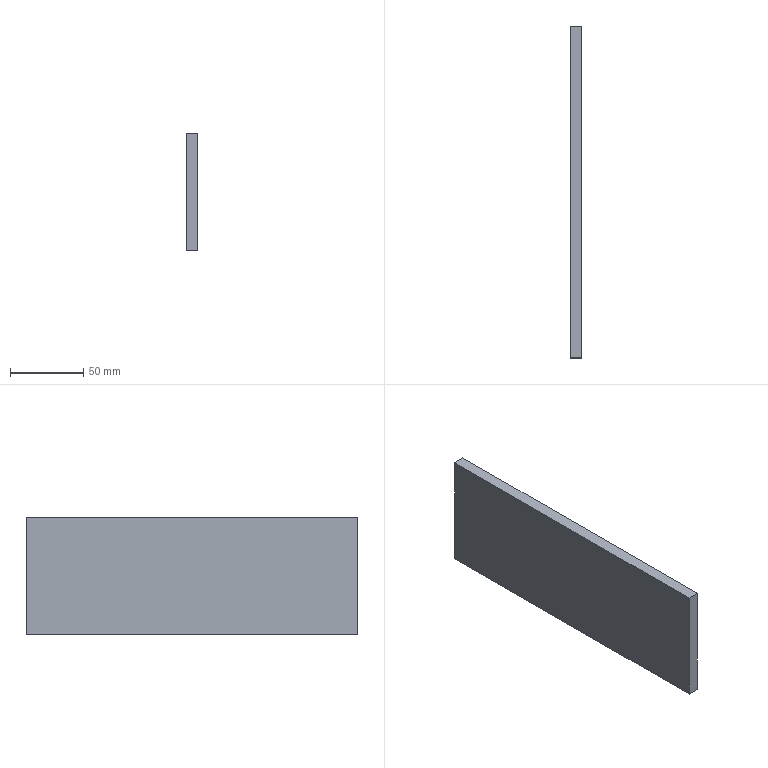Component | SolidWorks | RibPlate1-1 | 1 solid | 6 faces | box 8 x 226 x 80 mm | volume 144640 mm3 | plane 6 | material Plain Carbon Steel
STEP:
#1=CARTESIAN_POINT('',(17.897,53.911,65.555));
#2=VERTEX_POINT('',#1);
#3=CARTESIAN_POINT('',(17.897,53.911,68.704));
#4=VERTEX_POINT('',#3);
#5=CARTESIAN_POINT('',(17.897,53.911,68.704));
#6=DIRECTION('',(0.,-0.,1.));
#7=VECTOR('',#6,39.37);
#8=LINE('',#5,#7);
#9=EDGE_CURVE('',#2,#4,#8,.T.);
#10=ORIENTED_EDGE('',*,*,#9,.F.);
#11=CARTESIAN_POINT('',(17.582,53.911,65.555));
#12=VERTEX_POINT('',#11);
#13=CARTESIAN_POINT('',(17.582,53.911,65.555));
#14=DIRECTION('',(1.,0.,0.));
#15=VECTOR('',#14,39.37);
#16=LINE('',#13,#15);
#17=EDGE_CURVE('',#12,#2,#16,.T.);
#18=ORIENTED_EDGE('',*,*,#17,.F.);
#19=CARTESIAN_POINT('',(17.582,53.911,68.704));
#20=VERTEX_POINT('',#19);
#21=CARTESIAN_POINT('',(17.582,53.911,68.704));
#22=DIRECTION('',(0.,-0.,1.));
#23=VECTOR('',#22,39.37);
#24=LINE('',#21,#23);
#25=EDGE_CURVE('',#12,#20,#24,.T.);
#26=ORIENTED_EDGE('',*,*,#25,.T.);
#27=CARTESIAN_POINT('',(17.582,53.911,68.704));
#28=DIRECTION('',(1.,0.,0.));
#29=VECTOR('',#28,39.37);
#30=LINE('',#27,#29);
#31=EDGE_CURVE('',#20,#4,#30,.T.);
#32=ORIENTED_EDGE('',*,*,#31,.T.);
#33=EDGE_LOOP('',(#10,#18,#26,#32));
#34=FACE_OUTER_BOUND('',#33,.T.);
#35=CARTESIAN_POINT('',(17.582,53.911,68.704));
#36=DIRECTION('',(0.,1.,0.));
#37=DIRECTION('',(-1.,0.,0.));
#38=AXIS2_PLACEMENT_3D('',#35,#36,#37);
#39=PLANE('',#38);
#40=ADVANCED_FACE('',(#34),#39,.T.);
#41=CARTESIAN_POINT('',(17.897,45.014,65.555));
#42=VERTEX_POINT('',#41);
#43=CARTESIAN_POINT('',(17.897,45.014,65.555));
#44=DIRECTION('',(0.,1.,0.));
#45=VECTOR('',#44,39.37);
#46=LINE('',#43,#45);
#47=EDGE_CURVE('',#42,#2,#46,.T.);
#48=ORIENTED_EDGE('',*,*,#47,.F.);
#49=CARTESIAN_POINT('',(17.582,45.014,65.555));
#50=VERTEX_POINT('',#49);
#51=CARTESIAN_POINT('',(17.582,45.014,65.555));
#52=DIRECTION('',(1.,0.,0.));
#53=VECTOR('',#52,39.37);
#54=LINE('',#51,#53);
#55=EDGE_CURVE('',#50,#42,#54,.T.);
#56=ORIENTED_EDGE('',*,*,#55,.F.);
#57=CARTESIAN_POINT('',(17.582,45.014,65.555));
#58=DIRECTION('',(0.,1.,0.));
#59=VECTOR('',#58,39.37);
#60=LINE('',#57,#59);
#61=EDGE_CURVE('',#50,#12,#60,.T.);
#62=ORIENTED_EDGE('',*,*,#61,.T.);
#63=ORIENTED_EDGE('',*,*,#17,.T.);
#64=EDGE_LOOP('',(#48,#56,#62,#63));
#65=FACE_OUTER_BOUND('',#64,.T.);
#66=CARTESIAN_POINT('',(17.582,45.014,65.555));
#67=DIRECTION('',(0.,0.,-1.));
#68=DIRECTION('',(0.,1.,0.));
#69=AXIS2_PLACEMENT_3D('',#66,#67,#68);
#70=PLANE('',#69);
#71=ADVANCED_FACE('',(#65),#70,.T.);
#72=CARTESIAN_POINT('',(17.897,45.014,68.704));
#73=VERTEX_POINT('',#72);
#74=CARTESIAN_POINT('',(17.897,45.014,68.704));
#75=DIRECTION('',(0.,0.,-1.));
#76=VECTOR('',#75,39.37);
#77=LINE('',#74,#76);
#78=EDGE_CURVE('',#73,#42,#77,.T.);
#79=ORIENTED_EDGE('',*,*,#78,.F.);
#80=CARTESIAN_POINT('',(17.582,45.014,68.704));
#81=VERTEX_POINT('',#80);
#82=CARTESIAN_POINT('',(17.582,45.014,68.704));
#83=DIRECTION('',(1.,0.,0.));
#84=VECTOR('',#83,39.37);
#85=LINE('',#82,#84);
#86=EDGE_CURVE('',#81,#73,#85,.T.);
#87=ORIENTED_EDGE('',*,*,#86,.F.);
#88=CARTESIAN_POINT('',(17.582,45.014,68.704));
#89=DIRECTION('',(0.,0.,-1.));
#90=VECTOR('',#89,39.37);
#91=LINE('',#88,#90);
#92=EDGE_CURVE('',#81,#50,#91,.T.);
#93=ORIENTED_EDGE('',*,*,#92,.T.);
#94=ORIENTED_EDGE('',*,*,#55,.T.);
#95=EDGE_LOOP('',(#79,#87,#93,#94));
#96=FACE_OUTER_BOUND('',#95,.T.);
#97=CARTESIAN_POINT('',(17.582,45.014,68.704));
#98=DIRECTION('',(0.,-1.,-0.));
#99=DIRECTION('',(0.,0.,-1.));
#100=AXIS2_PLACEMENT_3D('',#97,#98,#99);
#101=PLANE('',#100);
#102=ADVANCED_FACE('',(#96),#101,.T.);
#103=CARTESIAN_POINT('',(17.897,45.014,68.704));
#104=DIRECTION('',(0.,-1.,-0.));
#105=VECTOR('',#104,39.37);
#106=LINE('',#103,#105);
#107=EDGE_CURVE('',#4,#73,#106,.T.);
#108=ORIENTED_EDGE('',*,*,#107,.F.);
#109=ORIENTED_EDGE('',*,*,#31,.F.);
#110=CARTESIAN_POINT('',(17.582,45.014,68.704));
#111=DIRECTION('',(0.,-1.,-0.));
#112=VECTOR('',#111,39.37);
#113=LINE('',#110,#112);
#114=EDGE_CURVE('',#20,#81,#113,.T.);
#115=ORIENTED_EDGE('',*,*,#114,.T.);
#116=ORIENTED_EDGE('',*,*,#86,.T.);
#117=EDGE_LOOP('',(#108,#109,#115,#116));
#118=FACE_OUTER_BOUND('',#117,.T.);
#119=CARTESIAN_POINT('',(17.582,45.014,68.704));
#120=DIRECTION('',(0.,-0.,1.));
#121=DIRECTION('',(0.,-1.,-0.));
#122=AXIS2_PLACEMENT_3D('',#119,#120,#121);
#123=PLANE('',#122);
#124=ADVANCED_FACE('',(#118),#123,.T.);
#125=ORIENTED_EDGE('',*,*,#25,.F.);
#126=ORIENTED_EDGE('',*,*,#61,.F.);
#127=ORIENTED_EDGE('',*,*,#92,.F.);
#128=ORIENTED_EDGE('',*,*,#114,.F.);
#129=EDGE_LOOP('',(#125,#126,#127,#128));
#130=FACE_OUTER_BOUND('',#129,.T.);
#131=CARTESIAN_POINT('',(17.582,49.134,62.367));
#132=DIRECTION('',(1.,0.,0.));
#133=DIRECTION('',(0.,1.,0.));
#134=AXIS2_PLACEMENT_3D('',#131,#132,#133);
#135=PLANE('',#134);
#136=ADVANCED_FACE('',(#130),#135,.F.);
#137=ORIENTED_EDGE('',*,*,#9,.T.);
#138=ORIENTED_EDGE('',*,*,#107,.T.);
#139=ORIENTED_EDGE('',*,*,#78,.T.);
#140=ORIENTED_EDGE('',*,*,#47,.T.);
#141=EDGE_LOOP('',(#137,#138,#139,#140));
#142=FACE_OUTER_BOUND('',#141,.T.);
#143=CARTESIAN_POINT('',(17.897,49.134,62.367));
#144=DIRECTION('',(1.,0.,0.));
#145=DIRECTION('',(0.,1.,0.));
#146=AXIS2_PLACEMENT_3D('',#143,#144,#145);
#147=PLANE('',#146);
#148=ADVANCED_FACE('',(#142),#147,.T.);
#149=CLOSED_SHELL('',(#40,#71,#102,#124,#136,#148));
#150=MANIFOLD_SOLID_BREP('',#149);
#151=CARTESIAN_POINT('',(0.,0.,0.));
#152=DIRECTION('',(0.,0.,1.));
#153=DIRECTION('',(1.,0.,0.));
#154=AXIS2_PLACEMENT_3D('',#151,#152,#153);
#155=(LENGTH_UNIT()NAMED_UNIT(*)SI_UNIT($,.METRE.));
#156=LENGTH_MEASURE_WITH_UNIT(LENGTH_MEASURE(0.0254),#155);
#157=DIMENSIONAL_EXPONENTS(1.,0.,0.,0.,0.,0.,0.);
#158=(CONVERSION_BASED_UNIT('',#156)LENGTH_UNIT()NAMED_UNIT(#157));
#159=UNCERTAINTY_MEASURE_WITH_UNIT(LENGTH_MEASURE(0.00001),#158,'','');
#160=(NAMED_UNIT(*)PLANE_ANGLE_UNIT()SI_UNIT($,.RADIAN.));
#161=(NAMED_UNIT(*)SI_UNIT($,.STERADIAN.)SOLID_ANGLE_UNIT());
#162=(GEOMETRIC_REPRESENTATION_CONTEXT(3)GLOBAL_UNCERTAINTY_ASSIGNED_CONTEXT((#159))GLOBAL_UNIT_ASSIGNED_CONTEXT((#158,#160,#161))REPRESENTATION_CONTEXT('',''));
#163=ADVANCED_BREP_SHAPE_REPRESENTATION('',(#150,#154),#162);
#164=COLOUR_RGB('',0.7922,0.8196,0.9333);
#165=FILL_AREA_STYLE_COLOUR('',#164);
#166=FILL_AREA_STYLE('',(#165));
#167=SURFACE_STYLE_FILL_AREA(#166);
#168=SURFACE_SIDE_STYLE('',(#167));
#169=SURFACE_STYLE_USAGE(.BOTH.,#168);
#170=PRESENTATION_STYLE_ASSIGNMENT((#169));
#171=STYLED_ITEM('',(#170),#150);
#172=(LENGTH_UNIT()NAMED_UNIT(*)SI_UNIT($,.METRE.));
#173=LENGTH_MEASURE_WITH_UNIT(LENGTH_MEASURE(0.0254),#172);
#174=DIMENSIONAL_EXPONENTS(1.,0.,0.,0.,0.,0.,0.);
#175=(CONVERSION_BASED_UNIT('',#173)LENGTH_UNIT()NAMED_UNIT(#174));
#176=UNCERTAINTY_MEASURE_WITH_UNIT(LENGTH_MEASURE(0.00001),#175,'','');
#177=(NAMED_UNIT(*)PLANE_ANGLE_UNIT()SI_UNIT($,.RADIAN.));
#178=(NAMED_UNIT(*)SI_UNIT($,.STERADIAN.)SOLID_ANGLE_UNIT());
#179=(GEOMETRIC_REPRESENTATION_CONTEXT(3)GLOBAL_UNCERTAINTY_ASSIGNED_CONTEXT((#176))GLOBAL_UNIT_ASSIGNED_CONTEXT((#175,#177,#178))REPRESENTATION_CONTEXT('',''));
#180=MECHANICAL_DESIGN_GEOMETRIC_PRESENTATION_REPRESENTATION('',(#171),#179);
#181=PRESENTATION_LAYER_ASSIGNMENT('','',(#171));